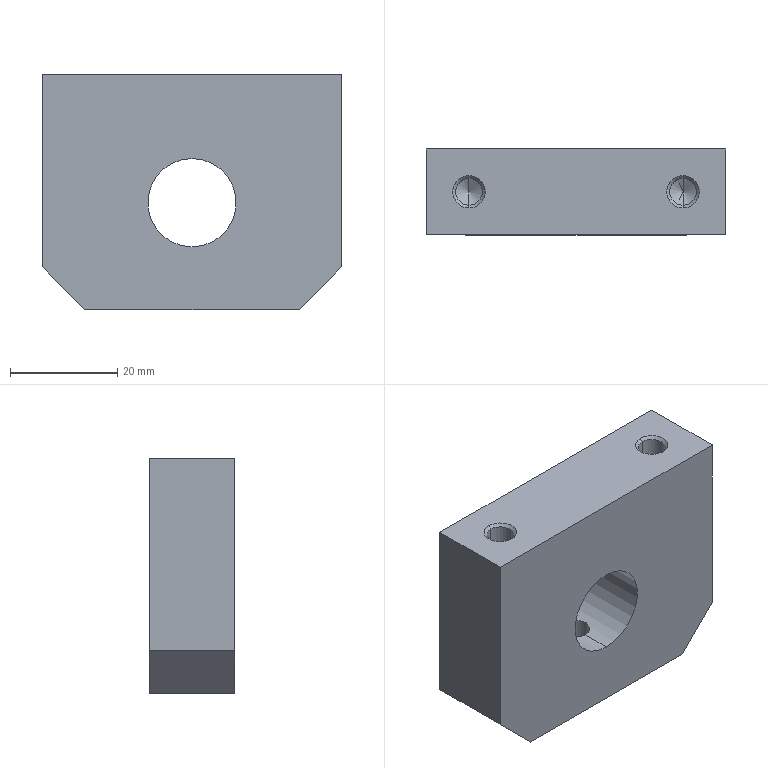Component | SolidWorks | GuideRodMount-2 | 1 solid | 26 faces | box 56 x 16 x 44 mm | volume 34052 mm3 | cone 10 | cylinder 8 | plane 8 | commonest cylinder face diameters 5 x6 16.5 x2
build123d program:
from build123d import *

# Parameters (mm, degrees)
SKETCH1_W                     = 44
SKETCH1_H                     = 56
BOSS_EXTRUDE1_DEPTH           = 16
F_16_5_16_5_DIAMETER_HOLE1_D  = 16.5
F_5_0_5_DIAMETER_HOLE1_REACH  = 54.764
F_5_0_5_DIAMETER_HOLE1_BORE_R = 2.5
F_5_0_5_DIAMETER_HOLE2_D      = 5
F_5_0_5_DIAMETER_HOLE2_DEPTH  = 17
F_5_0_5_DIAMETER_HOLE2_TIP    = 1.502
CHAMFER1_SIZE                 = 0.525
CHAMFER2_SIZE                 = 8


with BuildPart() as part:
    # Sketch1 → Boss-Extrude1 (new body)
    with BuildSketch(Plane(origin=(0, 0, -8), x_dir=(-1, 0, 0), z_dir=(0, 0, -1))):
        with Locations((-22, 0)):
            Rectangle(SKETCH1_W, SKETCH1_H)
    extrude(amount=-BOSS_EXTRUDE1_DEPTH)

    # 16.5 _16.5_ Diameter Hole1 (through all)
    with Locations(Plane.XY.offset(8)):
        with Locations((24, 0)):
            Hole(F_16_5_16_5_DIAMETER_HOLE1_D / 2)

    # 5.0 _5_ Diameter Hole1 bore → 5.0 _5_ Diameter Hole1 (cut, up to next)
    with BuildSketch(Plane(origin=(44, 0, 0), x_dir=(0, 0, -1), z_dir=(1, 0, 0)), mode=Mode.PRIVATE) as f_5_0_5_diameter_hole1_sk1:
        Circle(F_5_0_5_DIAMETER_HOLE1_BORE_R)
    f_5_0_5_diameter_hole1_tool1 = extrude(f_5_0_5_diameter_hole1_sk1.sketch, amount=-F_5_0_5_DIAMETER_HOLE1_REACH, mode=Mode.PRIVATE) & part.part
    add(f_5_0_5_diameter_hole1_tool1.solids().sort_by_distance((44, 0, 0))[0], mode=Mode.SUBTRACT)

    # 5.0 _5_ Diameter Hole2
    with Locations(Plane.ZY):
        with Locations((0, -20), (0, 20)):
            Hole(F_5_0_5_DIAMETER_HOLE2_D / 2, depth=F_5_0_5_DIAMETER_HOLE2_DEPTH)
            with Locations((0, 0, -(F_5_0_5_DIAMETER_HOLE2_DEPTH + F_5_0_5_DIAMETER_HOLE2_TIP / 2))):  # 118° drill point
                Cone(0, F_5_0_5_DIAMETER_HOLE2_D / 2, F_5_0_5_DIAMETER_HOLE2_TIP, mode=Mode.SUBTRACT)

    # Chamfer1
    chamfer1_edges = [part.edges().sort_by_distance(p)[0] for p in [
        (44, 0, 2.5),
        (0, 20, 2.5),
        (0, -20, 2.5),
    ]]
    chamfer(chamfer1_edges, length=CHAMFER1_SIZE)

    # Chamfer2
    chamfer2_edges = [part.edges().sort_by_distance(p)[0] for p in [
        (44, -28, 0),
        (44, 28, 0),
    ]]
    chamfer(chamfer2_edges, length=CHAMFER2_SIZE)


solid = part.part

# Placed as in the assembly
solid = solid.moved(Location((-36, -107, 262.5), (90, 0, -90)))
STEP:
#1=CARTESIAN_POINT('',(-0.6299,-4.114,10.314));
#2=VERTEX_POINT('',#1);
#3=CARTESIAN_POINT('',(-0.6299,-4.311,10.314));
#4=VERTEX_POINT('',#3);
#5=CARTESIAN_POINT('',(-0.6299,-4.213,10.314));
#6=DIRECTION('',(-0.,-0.,1.));
#7=DIRECTION('',(0.,-1.,0.));
#8=AXIS2_PLACEMENT_3D('',#5,#6,#7);
#9=CIRCLE('',#8,0.09843);
#10=EDGE_CURVE('',#2,#4,#9,.T.);
#11=ORIENTED_EDGE('',*,*,#10,.F.);
#12=CARTESIAN_POINT('',(-0.6299,-4.094,10.335));
#13=VERTEX_POINT('',#12);
#14=CARTESIAN_POINT('',(-0.6299,-4.114,10.314));
#15=DIRECTION('',(0.,0.7071,0.7071));
#16=VECTOR('',#15,39.37);
#17=LINE('',#14,#16);
#18=EDGE_CURVE('',#2,#13,#17,.T.);
#19=ORIENTED_EDGE('',*,*,#18,.T.);
#20=CARTESIAN_POINT('',(-0.6299,-4.332,10.335));
#21=VERTEX_POINT('',#20);
#22=CARTESIAN_POINT('',(-0.6299,-4.213,10.335));
#23=DIRECTION('',(0.,0.,-1.));
#24=DIRECTION('',(-1.,0.,0.));
#25=AXIS2_PLACEMENT_3D('',#22,#23,#24);
#26=CIRCLE('',#25,0.1191);
#27=EDGE_CURVE('',#21,#13,#26,.T.);
#28=ORIENTED_EDGE('',*,*,#27,.F.);
#29=CARTESIAN_POINT('',(-0.6299,-4.311,10.314));
#30=DIRECTION('',(0.,-0.7071,0.7071));
#31=VECTOR('',#30,39.37);
#32=LINE('',#29,#31);
#33=EDGE_CURVE('',#4,#21,#32,.T.);
#34=ORIENTED_EDGE('',*,*,#33,.F.);
#35=EDGE_LOOP('',(#11,#19,#28,#34));
#36=FACE_OUTER_BOUND('',#35,.T.);
#37=CARTESIAN_POINT('',(-0.6299,-4.213,10.314));
#38=DIRECTION('',(-0.,-0.,1.));
#39=DIRECTION('',(0.,-1.,0.));
#40=AXIS2_PLACEMENT_3D('',#37,#38,#39);
#41=CONICAL_SURFACE('',#40,0.09843,0.7854);
#42=ADVANCED_FACE('',(#36),#41,.F.);
#43=CARTESIAN_POINT('',(-2.205,-4.114,10.314));
#44=VERTEX_POINT('',#43);
#45=CARTESIAN_POINT('',(-2.205,-4.311,10.314));
#46=VERTEX_POINT('',#45);
#47=CARTESIAN_POINT('',(-2.205,-4.213,10.314));
#48=DIRECTION('',(-0.,-0.,1.));
#49=DIRECTION('',(0.,-1.,0.));
#50=AXIS2_PLACEMENT_3D('',#47,#48,#49);
#51=CIRCLE('',#50,0.09843);
#52=EDGE_CURVE('',#44,#46,#51,.T.);
#53=ORIENTED_EDGE('',*,*,#52,.F.);
#54=CARTESIAN_POINT('',(-2.205,-4.094,10.335));
#55=VERTEX_POINT('',#54);
#56=CARTESIAN_POINT('',(-2.205,-4.114,10.314));
#57=DIRECTION('',(0.,0.7071,0.7071));
#58=VECTOR('',#57,39.37);
#59=LINE('',#56,#58);
#60=EDGE_CURVE('',#44,#55,#59,.T.);
#61=ORIENTED_EDGE('',*,*,#60,.T.);
#62=CARTESIAN_POINT('',(-2.205,-4.332,10.335));
#63=VERTEX_POINT('',#62);
#64=CARTESIAN_POINT('',(-2.205,-4.213,10.335));
#65=DIRECTION('',(0.,0.,-1.));
#66=DIRECTION('',(-1.,0.,0.));
#67=AXIS2_PLACEMENT_3D('',#64,#65,#66);
#68=CIRCLE('',#67,0.1191);
#69=EDGE_CURVE('',#63,#55,#68,.T.);
#70=ORIENTED_EDGE('',*,*,#69,.F.);
#71=CARTESIAN_POINT('',(-2.205,-4.311,10.314));
#72=DIRECTION('',(0.,-0.7071,0.7071));
#73=VECTOR('',#72,39.37);
#74=LINE('',#71,#73);
#75=EDGE_CURVE('',#46,#63,#74,.T.);
#76=ORIENTED_EDGE('',*,*,#75,.F.);
#77=EDGE_LOOP('',(#53,#61,#70,#76));
#78=FACE_OUTER_BOUND('',#77,.T.);
#79=CARTESIAN_POINT('',(-2.205,-4.213,10.314));
#80=DIRECTION('',(-0.,-0.,1.));
#81=DIRECTION('',(0.,-1.,0.));
#82=AXIS2_PLACEMENT_3D('',#79,#80,#81);
#83=CONICAL_SURFACE('',#82,0.09843,0.7854);
#84=ADVANCED_FACE('',(#78),#83,.F.);
#85=CARTESIAN_POINT('',(-1.417,-4.311,8.623));
#86=VERTEX_POINT('',#85);
#87=CARTESIAN_POINT('',(-1.417,-4.114,8.623));
#88=VERTEX_POINT('',#87);
#89=CARTESIAN_POINT('',(-1.417,-4.213,8.623));
#90=DIRECTION('',(0.,0.,-1.));
#91=DIRECTION('',(0.,1.,0.));
#92=AXIS2_PLACEMENT_3D('',#89,#90,#91);
#93=CIRCLE('',#92,0.09843);
#94=EDGE_CURVE('',#86,#88,#93,.T.);
#95=ORIENTED_EDGE('',*,*,#94,.F.);
#96=CARTESIAN_POINT('',(-1.417,-4.332,8.602));
#97=VERTEX_POINT('',#96);
#98=CARTESIAN_POINT('',(-1.417,-4.311,8.623));
#99=DIRECTION('',(0.,-0.7071,-0.7071));
#100=VECTOR('',#99,39.37);
#101=LINE('',#98,#100);
#102=EDGE_CURVE('',#86,#97,#101,.T.);
#103=ORIENTED_EDGE('',*,*,#102,.T.);
#104=CARTESIAN_POINT('',(-1.417,-4.094,8.602));
#105=VERTEX_POINT('',#104);
#106=CARTESIAN_POINT('',(-1.417,-4.213,8.602));
#107=DIRECTION('',(-0.,-0.,1.));
#108=DIRECTION('',(0.,1.,0.));
#109=AXIS2_PLACEMENT_3D('',#106,#107,#108);
#110=CIRCLE('',#109,0.1191);
#111=EDGE_CURVE('',#105,#97,#110,.T.);
#112=ORIENTED_EDGE('',*,*,#111,.F.);
#113=CARTESIAN_POINT('',(-1.417,-4.114,8.623));
#114=DIRECTION('',(-0.,0.7071,-0.7071));
#115=VECTOR('',#114,39.37);
#116=LINE('',#113,#115);
#117=EDGE_CURVE('',#88,#105,#116,.T.);
#118=ORIENTED_EDGE('',*,*,#117,.F.);
#119=EDGE_LOOP('',(#95,#103,#112,#118));
#120=FACE_OUTER_BOUND('',#119,.T.);
#121=CARTESIAN_POINT('',(-1.417,-4.213,8.623));
#122=DIRECTION('',(0.,0.,-1.));
#123=DIRECTION('',(0.,1.,0.));
#124=AXIS2_PLACEMENT_3D('',#121,#122,#123);
#125=CONICAL_SURFACE('',#124,0.09843,0.7854);
#126=ADVANCED_FACE('',(#120),#125,.F.);
#127=CARTESIAN_POINT('',(-2.205,-4.114,9.665));
#128=VERTEX_POINT('',#127);
#129=CARTESIAN_POINT('',(-2.205,-4.311,9.665));
#130=VERTEX_POINT('',#129);
#131=CARTESIAN_POINT('',(-2.205,-4.213,9.665));
#132=DIRECTION('',(-0.,-0.,1.));
#133=DIRECTION('',(0.,-1.,0.));
#134=AXIS2_PLACEMENT_3D('',#131,#132,#133);
#135=CIRCLE('',#134,0.09843);
#136=EDGE_CURVE('',#128,#130,#135,.T.);
#137=ORIENTED_EDGE('',*,*,#136,.F.);
#138=CARTESIAN_POINT('',(-2.205,-4.114,10.335));
#139=DIRECTION('',(-0.,-0.,1.));
#140=VECTOR('',#139,39.37);
#141=LINE('',#138,#140);
#142=EDGE_CURVE('',#128,#44,#141,.T.);
#143=ORIENTED_EDGE('',*,*,#142,.T.);
#144=ORIENTED_EDGE('',*,*,#52,.T.);
#145=CARTESIAN_POINT('',(-2.205,-4.311,10.335));
#146=DIRECTION('',(-0.,-0.,1.));
#147=VECTOR('',#146,39.37);
#148=LINE('',#145,#147);
#149=EDGE_CURVE('',#130,#46,#148,.T.);
#150=ORIENTED_EDGE('',*,*,#149,.F.);
#151=EDGE_LOOP('',(#137,#143,#144,#150));
#152=FACE_OUTER_BOUND('',#151,.T.);
#153=CARTESIAN_POINT('',(-2.205,-4.213,10.335));
#154=DIRECTION('',(-0.,-0.,1.));
#155=DIRECTION('',(0.,-1.,0.));
#156=AXIS2_PLACEMENT_3D('',#153,#154,#155);
#157=CYLINDRICAL_SURFACE('',#156,0.09843);
#158=ADVANCED_FACE('',(#152),#157,.F.);
#159=CARTESIAN_POINT('',(-2.205,-4.213,9.606));
#160=VERTEX_POINT('',#159);
#161=CARTESIAN_POINT('',(-2.205,-4.311,9.665));
#162=DIRECTION('',(0.,-0.8572,0.515));
#163=VECTOR('',#162,39.37);
#164=LINE('',#161,#163);
#165=EDGE_CURVE('',#160,#130,#164,.T.);
#166=ORIENTED_EDGE('',*,*,#165,.F.);
#167=CARTESIAN_POINT('',(-2.205,-4.114,9.665));
#168=DIRECTION('',(0.,0.8572,0.515));
#169=VECTOR('',#168,39.37);
#170=LINE('',#167,#169);
#171=EDGE_CURVE('',#160,#128,#170,.T.);
#172=ORIENTED_EDGE('',*,*,#171,.T.);
#173=ORIENTED_EDGE('',*,*,#136,.T.);
#174=EDGE_LOOP('',(#166,#172,#173));
#175=FACE_OUTER_BOUND('',#174,.T.);
#176=CARTESIAN_POINT('',(-2.205,-4.213,9.665));
#177=DIRECTION('',(-0.,-0.,1.));
#178=DIRECTION('',(0.,-1.,0.));
#179=AXIS2_PLACEMENT_3D('',#176,#177,#178);
#180=CONICAL_SURFACE('',#179,0.09843,1.03);
#181=ADVANCED_FACE('',(#175),#180,.F.);
#182=CARTESIAN_POINT('',(-0.6299,-4.114,9.665));
#183=VERTEX_POINT('',#182);
#184=CARTESIAN_POINT('',(-0.6299,-4.311,9.665));
#185=VERTEX_POINT('',#184);
#186=CARTESIAN_POINT('',(-0.6299,-4.213,9.665));
#187=DIRECTION('',(-0.,-0.,1.));
#188=DIRECTION('',(0.,-1.,0.));
#189=AXIS2_PLACEMENT_3D('',#186,#187,#188);
#190=CIRCLE('',#189,0.09843);
#191=EDGE_CURVE('',#183,#185,#190,.T.);
#192=ORIENTED_EDGE('',*,*,#191,.F.);
#193=CARTESIAN_POINT('',(-0.6299,-4.114,10.335));
#194=DIRECTION('',(-0.,-0.,1.));
#195=VECTOR('',#194,39.37);
#196=LINE('',#193,#195);
#197=EDGE_CURVE('',#183,#2,#196,.T.);
#198=ORIENTED_EDGE('',*,*,#197,.T.);
#199=ORIENTED_EDGE('',*,*,#10,.T.);
#200=CARTESIAN_POINT('',(-0.6299,-4.311,10.335));
#201=DIRECTION('',(-0.,-0.,1.));
#202=VECTOR('',#201,39.37);
#203=LINE('',#200,#202);
#204=EDGE_CURVE('',#185,#4,#203,.T.);
#205=ORIENTED_EDGE('',*,*,#204,.F.);
#206=EDGE_LOOP('',(#192,#198,#199,#205));
#207=FACE_OUTER_BOUND('',#206,.T.);
#208=CARTESIAN_POINT('',(-0.6299,-4.213,10.335));
#209=DIRECTION('',(-0.,-0.,1.));
#210=DIRECTION('',(0.,-1.,0.));
#211=AXIS2_PLACEMENT_3D('',#208,#209,#210);
#212=CYLINDRICAL_SURFACE('',#211,0.09843);
#213=ADVANCED_FACE('',(#207),#212,.F.);
#214=CARTESIAN_POINT('',(-0.6299,-4.213,9.606));
#215=VERTEX_POINT('',#214);
#216=CARTESIAN_POINT('',(-0.6299,-4.311,9.665));
#217=DIRECTION('',(0.,-0.8572,0.515));
#218=VECTOR('',#217,39.37);
#219=LINE('',#216,#218);
#220=EDGE_CURVE('',#215,#185,#219,.T.);
#221=ORIENTED_EDGE('',*,*,#220,.F.);
#222=CARTESIAN_POINT('',(-0.6299,-4.114,9.665));
#223=DIRECTION('',(0.,0.8572,0.515));
#224=VECTOR('',#223,39.37);
#225=LINE('',#222,#224);
#226=EDGE_CURVE('',#215,#183,#225,.T.);
#227=ORIENTED_EDGE('',*,*,#226,.T.);
#228=ORIENTED_EDGE('',*,*,#191,.T.);
#229=EDGE_LOOP('',(#221,#227,#228));
#230=FACE_OUTER_BOUND('',#229,.T.);
#231=CARTESIAN_POINT('',(-0.6299,-4.213,9.665));
#232=DIRECTION('',(-0.,-0.,1.));
#233=DIRECTION('',(0.,-1.,0.));
#234=AXIS2_PLACEMENT_3D('',#231,#232,#233);
#235=CONICAL_SURFACE('',#234,0.09843,1.03);
#236=ADVANCED_FACE('',(#230),#235,.F.);
#237=CARTESIAN_POINT('',(-1.417,-4.311,9.065));
#238=VERTEX_POINT('',#237);
#239=CARTESIAN_POINT('',(-1.417,-4.114,9.065));
#240=VERTEX_POINT('',#239);
#241=CARTESIAN_POINT('',(-1.417,-4.311,9.065));
#242=CARTESIAN_POINT('',(-1.43,-4.311,9.065));
#243=CARTESIAN_POINT('',(-1.443,-4.308,9.066));
#244=CARTESIAN_POINT('',(-1.461,-4.301,9.068));
#245=CARTESIAN_POINT('',(-1.467,-4.298,9.069));
#246=CARTESIAN_POINT('',(-1.477,-4.291,9.071));
#247=CARTESIAN_POINT('',(-1.482,-4.287,9.072));
#248=CARTESIAN_POINT('',(-1.491,-4.278,9.073));
#249=CARTESIAN_POINT('',(-1.496,-4.273,9.075));
#250=CARTESIAN_POINT('',(-1.503,-4.262,9.076));
#251=CARTESIAN_POINT('',(-1.506,-4.256,9.077));
#252=CARTESIAN_POINT('',(-1.511,-4.244,9.079));
#253=CARTESIAN_POINT('',(-1.513,-4.238,9.079));
#254=CARTESIAN_POINT('',(-1.515,-4.226,9.08));
#255=CARTESIAN_POINT('',(-1.516,-4.219,9.08));
#256=CARTESIAN_POINT('',(-1.516,-4.206,9.08));
#257=CARTESIAN_POINT('',(-1.515,-4.2,9.08));
#258=CARTESIAN_POINT('',(-1.513,-4.187,9.079));
#259=CARTESIAN_POINT('',(-1.511,-4.181,9.079));
#260=CARTESIAN_POINT('',(-1.503,-4.163,9.076));
#261=CARTESIAN_POINT('',(-1.496,-4.152,9.074));
#262=CARTESIAN_POINT('',(-1.482,-4.139,9.072));
#263=CARTESIAN_POINT('',(-1.477,-4.134,9.071));
#264=CARTESIAN_POINT('',(-1.467,-4.127,9.069));
#265=CARTESIAN_POINT('',(-1.461,-4.124,9.068));
#266=CARTESIAN_POINT('',(-1.449,-4.119,9.066));
#267=CARTESIAN_POINT('',(-1.443,-4.117,9.066));
#268=CARTESIAN_POINT('',(-1.43,-4.115,9.065));
#269=CARTESIAN_POINT('',(-1.424,-4.114,9.065));
#270=CARTESIAN_POINT('',(-1.417,-4.114,9.065));
#271=B_SPLINE_CURVE_WITH_KNOTS('',3,(#241,#242,#243,#244,#245,#246,#247,#248,#249,#250,#251,#252,#253,#254,#255,#256,#257,#258,#259,#260,#261,#262,#263,#264,#265,#266,#267,#268,#269,#270),.UNSPECIFIED.,.F.,.F.,(4,2,2,2,2,2,2,2,2,2,2,2,2,2,4),(0.007863,0.008845,0.009336,0.009828,0.01032,0.01081,0.0113,0.01179,0.01228,0.01278,0.01376,0.01425,0.01474,0.01523,0.01572),.UNSPECIFIED.);
#272=EDGE_CURVE('',#238,#240,#271,.T.);
#273=ORIENTED_EDGE('',*,*,#272,.F.);
#274=CARTESIAN_POINT('',(-1.417,-4.311,8.602));
#275=DIRECTION('',(0.,0.,-1.));
#276=VECTOR('',#275,39.37);
#277=LINE('',#274,#276);
#278=EDGE_CURVE('',#238,#86,#277,.T.);
#279=ORIENTED_EDGE('',*,*,#278,.T.);
#280=ORIENTED_EDGE('',*,*,#94,.T.);
#281=CARTESIAN_POINT('',(-1.417,-4.114,8.602));
#282=DIRECTION('',(0.,0.,-1.));
#283=VECTOR('',#282,39.37);
#284=LINE('',#281,#283);
#285=EDGE_CURVE('',#240,#88,#284,.T.);
#286=ORIENTED_EDGE('',*,*,#285,.F.);
#287=EDGE_LOOP('',(#273,#279,#280,#286));
#288=FACE_OUTER_BOUND('',#287,.T.);
#289=CARTESIAN_POINT('',(-1.417,-4.213,8.602));
#290=DIRECTION('',(0.,0.,-1.));
#291=DIRECTION('',(0.,1.,0.));
#292=AXIS2_PLACEMENT_3D('',#289,#290,#291);
#293=CYLINDRICAL_SURFACE('',#292,0.09843);
#294=ADVANCED_FACE('',(#288),#293,.F.);
#295=CARTESIAN_POINT('',(-1.417,-3.898,9.715));
#296=VERTEX_POINT('',#295);
#297=CARTESIAN_POINT('',(-1.417,-3.898,9.065));
#298=VERTEX_POINT('',#297);
#299=CARTESIAN_POINT('',(-1.417,-3.898,9.39));
#300=DIRECTION('',(0.,-1.,0.));
#301=DIRECTION('',(0.,0.,-1.));
#302=AXIS2_PLACEMENT_3D('',#299,#300,#301);
#303=CIRCLE('',#302,0.3248);
#304=EDGE_CURVE('',#296,#298,#303,.T.);
#305=ORIENTED_EDGE('',*,*,#304,.F.);
#306=CARTESIAN_POINT('',(-1.417,-4.528,9.715));
#307=VERTEX_POINT('',#306);
#308=CARTESIAN_POINT('',(-1.417,-4.528,9.715));
#309=DIRECTION('',(0.,-1.,0.));
#310=VECTOR('',#309,39.37);
#311=LINE('',#308,#310);
#312=EDGE_CURVE('',#296,#307,#311,.T.);
#313=ORIENTED_EDGE('',*,*,#312,.T.);
#314=CARTESIAN_POINT('',(-1.417,-4.528,9.065));
#315=VERTEX_POINT('',#314);
#316=CARTESIAN_POINT('',(-1.417,-4.528,9.39));
#317=DIRECTION('',(0.,-1.,0.));
#318=DIRECTION('',(0.,0.,-1.));
#319=AXIS2_PLACEMENT_3D('',#316,#317,#318);
#320=CIRCLE('',#319,0.3248);
#321=EDGE_CURVE('',#307,#315,#320,.T.);
#322=ORIENTED_EDGE('',*,*,#321,.T.);
#323=CARTESIAN_POINT('',(-1.417,-4.528,9.065));
#324=DIRECTION('',(0.,-1.,0.));
#325=VECTOR('',#324,39.37);
#326=LINE('',#323,#325);
#327=EDGE_CURVE('',#238,#315,#326,.T.);
#328=ORIENTED_EDGE('',*,*,#327,.F.);
#329=ORIENTED_EDGE('',*,*,#272,.T.);
#330=CARTESIAN_POINT('',(-1.417,-4.528,9.065));
#331=DIRECTION('',(0.,-1.,0.));
#332=VECTOR('',#331,39.37);
#333=LINE('',#330,#332);
#334=EDGE_CURVE('',#298,#240,#333,.T.);
#335=ORIENTED_EDGE('',*,*,#334,.F.);
#336=EDGE_LOOP('',(#305,#313,#322,#328,#329,#335));
#337=FACE_OUTER_BOUND('',#336,.T.);
#338=CARTESIAN_POINT('',(-1.417,-4.528,9.39));
#339=DIRECTION('',(0.,-1.,0.));
#340=DIRECTION('',(0.,0.,-1.));
#341=AXIS2_PLACEMENT_3D('',#338,#339,#340);
#342=CYLINDRICAL_SURFACE('',#341,0.3248);
#343=ADVANCED_FACE('',(#337),#342,.F.);
#344=CARTESIAN_POINT('',(-0.315,-4.528,10.335));
#345=VERTEX_POINT('',#344);
#346=CARTESIAN_POINT('',(-0.315,-4.528,8.917));
#347=VERTEX_POINT('',#346);
#348=CARTESIAN_POINT('',(-0.315,-4.528,10.335));
#349=DIRECTION('',(0.,0.,-1.));
#350=VECTOR('',#349,39.37);
#351=LINE('',#348,#350);
#352=EDGE_CURVE('',#345,#347,#351,.T.);
#353=ORIENTED_EDGE('',*,*,#352,.T.);
#354=CARTESIAN_POINT('',(-0.315,-3.898,8.917));
#355=VERTEX_POINT('',#354);
#356=CARTESIAN_POINT('',(-0.315,-4.528,8.917));
#357=DIRECTION('',(-0.,1.,0.));
#358=VECTOR('',#357,39.37);
#359=LINE('',#356,#358);
#360=EDGE_CURVE('',#347,#355,#359,.T.);
#361=ORIENTED_EDGE('',*,*,#360,.T.);
#362=CARTESIAN_POINT('',(-0.315,-3.898,10.335));
#363=VERTEX_POINT('',#362);
#364=CARTESIAN_POINT('',(-0.315,-3.898,10.335));
#365=DIRECTION('',(0.,0.,-1.));
#366=VECTOR('',#365,39.37);
#367=LINE('',#364,#366);
#368=EDGE_CURVE('',#363,#355,#367,.T.);
#369=ORIENTED_EDGE('',*,*,#368,.F.);
#370=CARTESIAN_POINT('',(-0.315,-4.528,10.335));
#371=DIRECTION('',(-0.,1.,0.));
#372=VECTOR('',#371,39.37);
#373=LINE('',#370,#372);
#374=EDGE_CURVE('',#345,#363,#373,.T.);
#375=ORIENTED_EDGE('',*,*,#374,.F.);
#376=EDGE_LOOP('',(#353,#361,#369,#375));
#377=FACE_OUTER_BOUND('',#376,.T.);
#378=CARTESIAN_POINT('',(-0.315,-4.528,10.335));
#379=DIRECTION('',(1.,0.,0.));
#380=DIRECTION('',(0.,-1.,0.));
#381=AXIS2_PLACEMENT_3D('',#378,#379,#380);
#382=PLANE('',#381);
#383=ADVANCED_FACE('',(#377),#382,.T.);
#384=ORIENTED_EDGE('',*,*,#69,.T.);
#385=CARTESIAN_POINT('',(-2.205,-4.213,10.335));
#386=DIRECTION('',(0.,0.,-1.));
#387=DIRECTION('',(-1.,0.,0.));
#388=AXIS2_PLACEMENT_3D('',#385,#386,#387);
#389=CIRCLE('',#388,0.1191);
#390=EDGE_CURVE('',#55,#63,#389,.T.);
#391=ORIENTED_EDGE('',*,*,#390,.T.);
#392=EDGE_LOOP('',(#384,#391));
#393=FACE_BOUND('',#392,.T.);
#394=ORIENTED_EDGE('',*,*,#27,.T.);
#395=CARTESIAN_POINT('',(-0.6299,-4.213,10.335));
#396=DIRECTION('',(0.,0.,-1.));
#397=DIRECTION('',(-1.,0.,0.));
#398=AXIS2_PLACEMENT_3D('',#395,#396,#397);
#399=CIRCLE('',#398,0.1191);
#400=EDGE_CURVE('',#13,#21,#399,.T.);
#401=ORIENTED_EDGE('',*,*,#400,.T.);
#402=EDGE_LOOP('',(#394,#401));
#403=FACE_BOUND('',#402,.T.);
#404=CARTESIAN_POINT('',(-2.52,-3.898,10.335));
#405=VERTEX_POINT('',#404);
#406=CARTESIAN_POINT('',(-2.52,-3.898,10.335));
#407=DIRECTION('',(1.,0.,0.));
#408=VECTOR('',#407,39.37);
#409=LINE('',#406,#408);
#410=EDGE_CURVE('',#405,#363,#409,.T.);
#411=ORIENTED_EDGE('',*,*,#410,.F.);
#412=CARTESIAN_POINT('',(-2.52,-4.528,10.335));
#413=VERTEX_POINT('',#412);
#414=CARTESIAN_POINT('',(-2.52,-4.528,10.335));
#415=DIRECTION('',(-0.,1.,0.));
#416=VECTOR('',#415,39.37);
#417=LINE('',#414,#416);
#418=EDGE_CURVE('',#413,#405,#417,.T.);
#419=ORIENTED_EDGE('',*,*,#418,.F.);
#420=CARTESIAN_POINT('',(-2.52,-4.528,10.335));
#421=DIRECTION('',(1.,0.,0.));
#422=VECTOR('',#421,39.37);
#423=LINE('',#420,#422);
#424=EDGE_CURVE('',#413,#345,#423,.T.);
#425=ORIENTED_EDGE('',*,*,#424,.T.);
#426=ORIENTED_EDGE('',*,*,#374,.T.);
#427=EDGE_LOOP('',(#411,#419,#425,#426));
#428=FACE_OUTER_BOUND('',#427,.T.);
#429=CARTESIAN_POINT('',(-2.52,-4.528,10.335));
#430=DIRECTION('',(-0.,-0.,1.));
#431=DIRECTION('',(-1.,-0.,-0.));
#432=AXIS2_PLACEMENT_3D('',#429,#430,#431);
#433=PLANE('',#432);
#434=ADVANCED_FACE('',(#393,#403,#428),#433,.T.);
#435=CARTESIAN_POINT('',(-2.52,-3.898,8.917));
#436=VERTEX_POINT('',#435);
#437=CARTESIAN_POINT('',(-2.52,-3.898,8.602));
#438=DIRECTION('',(-0.,-0.,1.));
#439=VECTOR('',#438,39.37);
#440=LINE('',#437,#439);
#441=EDGE_CURVE('',#436,#405,#440,.T.);
#442=ORIENTED_EDGE('',*,*,#441,.F.);
#443=CARTESIAN_POINT('',(-2.52,-4.528,8.917));
#444=VERTEX_POINT('',#443);
#445=CARTESIAN_POINT('',(-2.52,-4.528,8.917));
#446=DIRECTION('',(0.,-1.,0.));
#447=VECTOR('',#446,39.37);
#448=LINE('',#445,#447);
#449=EDGE_CURVE('',#436,#444,#448,.T.);
#450=ORIENTED_EDGE('',*,*,#449,.T.);
#451=CARTESIAN_POINT('',(-2.52,-4.528,8.602));
#452=DIRECTION('',(-0.,-0.,1.));
#453=VECTOR('',#452,39.37);
#454=LINE('',#451,#453);
#455=EDGE_CURVE('',#444,#413,#454,.T.);
#456=ORIENTED_EDGE('',*,*,#455,.T.);
#457=ORIENTED_EDGE('',*,*,#418,.T.);
#458=EDGE_LOOP('',(#442,#450,#456,#457));
#459=FACE_OUTER_BOUND('',#458,.T.);
#460=CARTESIAN_POINT('',(-2.52,-4.528,8.602));
#461=DIRECTION('',(-1.,-0.,-0.));
#462=DIRECTION('',(-0.,1.,0.));
#463=AXIS2_PLACEMENT_3D('',#460,#461,#462);
#464=PLANE('',#463);
#465=ADVANCED_FACE('',(#459),#464,.T.);
#466=ORIENTED_EDGE('',*,*,#111,.T.);
#467=CARTESIAN_POINT('',(-1.417,-4.213,8.602));
#468=DIRECTION('',(-0.,-0.,1.));
#469=DIRECTION('',(0.,1.,0.));
#470=AXIS2_PLACEMENT_3D('',#467,#468,#469);
#471=CIRCLE('',#470,0.1191);
#472=EDGE_CURVE('',#97,#105,#471,.T.);
#473=ORIENTED_EDGE('',*,*,#472,.T.);
#474=EDGE_LOOP('',(#466,#473));
#475=FACE_BOUND('',#474,.T.);
#476=CARTESIAN_POINT('',(-0.6299,-3.898,8.602));
#477=VERTEX_POINT('',#476);
#478=CARTESIAN_POINT('',(-2.205,-3.898,8.602));
#479=VERTEX_POINT('',#478);
#480=CARTESIAN_POINT('',(-0.315,-3.898,8.602));
#481=DIRECTION('',(-1.,-0.,-0.));
#482=VECTOR('',#481,39.37);
#483=LINE('',#480,#482);
#484=EDGE_CURVE('',#477,#479,#483,.T.);
#485=ORIENTED_EDGE('',*,*,#484,.F.);
#486=CARTESIAN_POINT('',(-0.6299,-4.528,8.602));
#487=VERTEX_POINT('',#486);
#488=CARTESIAN_POINT('',(-0.6299,-4.528,8.602));
#489=DIRECTION('',(0.,-1.,0.));
#490=VECTOR('',#489,39.37);
#491=LINE('',#488,#490);
#492=EDGE_CURVE('',#477,#487,#491,.T.);
#493=ORIENTED_EDGE('',*,*,#492,.T.);
#494=CARTESIAN_POINT('',(-2.205,-4.528,8.602));
#495=VERTEX_POINT('',#494);
#496=CARTESIAN_POINT('',(-0.315,-4.528,8.602));
#497=DIRECTION('',(-1.,-0.,-0.));
#498=VECTOR('',#497,39.37);
#499=LINE('',#496,#498);
#500=EDGE_CURVE('',#487,#495,#499,.T.);
#501=ORIENTED_EDGE('',*,*,#500,.T.);
#502=CARTESIAN_POINT('',(-2.205,-4.528,8.602));
#503=DIRECTION('',(-0.,1.,0.));
#504=VECTOR('',#503,39.37);
#505=LINE('',#502,#504);
#506=EDGE_CURVE('',#495,#479,#505,.T.);
#507=ORIENTED_EDGE('',*,*,#506,.T.);
#508=EDGE_LOOP('',(#485,#493,#501,#507));
#509=FACE_OUTER_BOUND('',#508,.T.);
#510=CARTESIAN_POINT('',(-0.315,-4.528,8.602));
#511=DIRECTION('',(0.,0.,-1.));
#512=DIRECTION('',(-0.,1.,0.));
#513=AXIS2_PLACEMENT_3D('',#510,#511,#512);
#514=PLANE('',#513);
#515=ADVANCED_FACE('',(#475,#509),#514,.T.);
#516=CARTESIAN_POINT('',(-1.417,-4.528,9.39));
#517=DIRECTION('',(0.,-1.,0.));
#518=DIRECTION('',(0.,0.,-1.));
#519=AXIS2_PLACEMENT_3D('',#516,#517,#518);
#520=CIRCLE('',#519,0.3248);
#521=EDGE_CURVE('',#315,#307,#520,.T.);
#522=ORIENTED_EDGE('',*,*,#521,.F.);
#523=ORIENTED_EDGE('',*,*,#321,.F.);
#524=EDGE_LOOP('',(#522,#523));
#525=FACE_BOUND('',#524,.T.);
#526=ORIENTED_EDGE('',*,*,#500,.F.);
#527=CARTESIAN_POINT('',(-0.315,-4.528,8.917));
#528=DIRECTION('',(0.7071,0.,0.7071));
#529=VECTOR('',#528,39.37);
#530=LINE('',#527,#529);
#531=EDGE_CURVE('',#487,#347,#530,.T.);
#532=ORIENTED_EDGE('',*,*,#531,.T.);
#533=ORIENTED_EDGE('',*,*,#352,.F.);
#534=ORIENTED_EDGE('',*,*,#424,.F.);
#535=ORIENTED_EDGE('',*,*,#455,.F.);
#536=CARTESIAN_POINT('',(-2.205,-4.528,8.602));
#537=DIRECTION('',(0.7071,0.,-0.7071));
#538=VECTOR('',#537,39.37);
#539=LINE('',#536,#538);
#540=EDGE_CURVE('',#444,#495,#539,.T.);
#541=ORIENTED_EDGE('',*,*,#540,.T.);
#542=EDGE_LOOP('',(#526,#532,#533,#534,#535,#541));
#543=FACE_OUTER_BOUND('',#542,.T.);
#544=CARTESIAN_POINT('',(-1.417,-4.528,10.335));
#545=DIRECTION('',(-0.,1.,0.));
#546=DIRECTION('',(-0.,-0.,1.));
#547=AXIS2_PLACEMENT_3D('',#544,#545,#546);
#548=PLANE('',#547);
#549=ADVANCED_FACE('',(#525,#543),#548,.F.);
#550=CARTESIAN_POINT('',(-1.417,-3.898,9.39));
#551=DIRECTION('',(0.,-1.,0.));
#552=DIRECTION('',(0.,0.,-1.));
#553=AXIS2_PLACEMENT_3D('',#550,#551,#552);
#554=CIRCLE('',#553,0.3248);
#555=EDGE_CURVE('',#298,#296,#554,.T.);
#556=ORIENTED_EDGE('',*,*,#555,.T.);
#557=ORIENTED_EDGE('',*,*,#304,.T.);
#558=EDGE_LOOP('',(#556,#557));
#559=FACE_BOUND('',#558,.T.);
#560=ORIENTED_EDGE('',*,*,#368,.T.);
#561=CARTESIAN_POINT('',(-0.1575,-3.898,9.075));
#562=DIRECTION('',(-0.7071,-0.,-0.7071));
#563=VECTOR('',#562,39.37);
#564=LINE('',#561,#563);
#565=EDGE_CURVE('',#355,#477,#564,.T.);
#566=ORIENTED_EDGE('',*,*,#565,.T.);
#567=ORIENTED_EDGE('',*,*,#484,.T.);
#568=CARTESIAN_POINT('',(-2.677,-3.898,9.075));
#569=DIRECTION('',(-0.7071,-0.,0.7071));
#570=VECTOR('',#569,39.37);
#571=LINE('',#568,#570);
#572=EDGE_CURVE('',#479,#436,#571,.T.);
#573=ORIENTED_EDGE('',*,*,#572,.T.);
#574=ORIENTED_EDGE('',*,*,#441,.T.);
#575=ORIENTED_EDGE('',*,*,#410,.T.);
#576=EDGE_LOOP('',(#560,#566,#567,#573,#574,#575));
#577=FACE_OUTER_BOUND('',#576,.T.);
#578=CARTESIAN_POINT('',(-1.417,-3.898,10.335));
#579=DIRECTION('',(-0.,1.,0.));
#580=DIRECTION('',(-0.,-0.,1.));
#581=AXIS2_PLACEMENT_3D('',#578,#579,#580);
#582=PLANE('',#581);
#583=ADVANCED_FACE('',(#559,#577),#582,.T.);
#584=ORIENTED_EDGE('',*,*,#312,.F.);
#585=ORIENTED_EDGE('',*,*,#555,.F.);
#586=ORIENTED_EDGE('',*,*,#334,.T.);
#587=CARTESIAN_POINT('',(-1.417,-4.114,9.065));
#588=CARTESIAN_POINT('',(-1.411,-4.114,9.065));
#589=CARTESIAN_POINT('',(-1.404,-4.115,9.065));
#590=CARTESIAN_POINT('',(-1.392,-4.117,9.066));
#591=CARTESIAN_POINT('',(-1.385,-4.119,9.066));
#592=CARTESIAN_POINT('',(-1.374,-4.124,9.068));
#593=CARTESIAN_POINT('',(-1.368,-4.127,9.069));
#594=CARTESIAN_POINT('',(-1.357,-4.134,9.071));
#595=CARTESIAN_POINT('',(-1.352,-4.139,9.072));
#596=CARTESIAN_POINT('',(-1.339,-4.152,9.074));
#597=CARTESIAN_POINT('',(-1.331,-4.163,9.076));
#598=CARTESIAN_POINT('',(-1.324,-4.181,9.079));
#599=CARTESIAN_POINT('',(-1.322,-4.187,9.079));
#600=CARTESIAN_POINT('',(-1.32,-4.2,9.08));
#601=CARTESIAN_POINT('',(-1.319,-4.206,9.08));
#602=CARTESIAN_POINT('',(-1.319,-4.219,9.08));
#603=CARTESIAN_POINT('',(-1.32,-4.226,9.08));
#604=CARTESIAN_POINT('',(-1.322,-4.238,9.079));
#605=CARTESIAN_POINT('',(-1.324,-4.244,9.079));
#606=CARTESIAN_POINT('',(-1.329,-4.256,9.077));
#607=CARTESIAN_POINT('',(-1.332,-4.262,9.076));
#608=CARTESIAN_POINT('',(-1.339,-4.273,9.075));
#609=CARTESIAN_POINT('',(-1.343,-4.278,9.073));
#610=CARTESIAN_POINT('',(-1.352,-4.287,9.072));
#611=CARTESIAN_POINT('',(-1.357,-4.291,9.071));
#612=CARTESIAN_POINT('',(-1.368,-4.298,9.069));
#613=CARTESIAN_POINT('',(-1.374,-4.301,9.068));
#614=CARTESIAN_POINT('',(-1.385,-4.306,9.066));
#615=CARTESIAN_POINT('',(-1.392,-4.308,9.066));
#616=CARTESIAN_POINT('',(-1.404,-4.31,9.065));
#617=CARTESIAN_POINT('',(-1.411,-4.311,9.065));
#618=CARTESIAN_POINT('',(-1.417,-4.311,9.065));
#619=B_SPLINE_CURVE_WITH_KNOTS('',3,(#587,#588,#589,#590,#591,#592,#593,#594,#595,#596,#597,#598,#599,#600,#601,#602,#603,#604,#605,#606,#607,#608,#609,#610,#611,#612,#613,#614,#615,#616,#617,#618),.UNSPECIFIED.,.F.,.F.,(4,2,2,2,2,2,2,2,2,2,2,2,2,2,2,4),(0.,0.0004914,0.0009828,0.001474,0.001966,0.002948,0.00344,0.003931,0.004423,0.004914,0.005406,0.005897,0.006388,0.00688,0.007371,0.007863),.UNSPECIFIED.);
#620=EDGE_CURVE('',#240,#238,#619,.T.);
#621=ORIENTED_EDGE('',*,*,#620,.T.);
#622=ORIENTED_EDGE('',*,*,#327,.T.);
#623=ORIENTED_EDGE('',*,*,#521,.T.);
#624=EDGE_LOOP('',(#584,#585,#586,#621,#622,#623));
#625=FACE_OUTER_BOUND('',#624,.T.);
#626=CARTESIAN_POINT('',(-1.417,-4.528,9.39));
#627=DIRECTION('',(0.,-1.,0.));
#628=DIRECTION('',(0.,0.,-1.));
#629=AXIS2_PLACEMENT_3D('',#626,#627,#628);
#630=CYLINDRICAL_SURFACE('',#629,0.3248);
#631=ADVANCED_FACE('',(#625),#630,.F.);
#632=ORIENTED_EDGE('',*,*,#278,.F.);
#633=ORIENTED_EDGE('',*,*,#620,.F.);
#634=ORIENTED_EDGE('',*,*,#285,.T.);
#635=CARTESIAN_POINT('',(-1.417,-4.213,8.623));
#636=DIRECTION('',(0.,0.,-1.));
#637=DIRECTION('',(0.,1.,0.));
#638=AXIS2_PLACEMENT_3D('',#635,#636,#637);
#639=CIRCLE('',#638,0.09843);
#640=EDGE_CURVE('',#88,#86,#639,.T.);
#641=ORIENTED_EDGE('',*,*,#640,.T.);
#642=EDGE_LOOP('',(#632,#633,#634,#641));
#643=FACE_OUTER_BOUND('',#642,.T.);
#644=CARTESIAN_POINT('',(-1.417,-4.213,8.602));
#645=DIRECTION('',(0.,0.,-1.));
#646=DIRECTION('',(0.,1.,0.));
#647=AXIS2_PLACEMENT_3D('',#644,#645,#646);
#648=CYLINDRICAL_SURFACE('',#647,0.09843);
#649=ADVANCED_FACE('',(#643),#648,.F.);
#650=ORIENTED_EDGE('',*,*,#226,.F.);
#651=ORIENTED_EDGE('',*,*,#220,.T.);
#652=CARTESIAN_POINT('',(-0.6299,-4.213,9.665));
#653=DIRECTION('',(-0.,-0.,1.));
#654=DIRECTION('',(0.,-1.,0.));
#655=AXIS2_PLACEMENT_3D('',#652,#653,#654);
#656=CIRCLE('',#655,0.09843);
#657=EDGE_CURVE('',#185,#183,#656,.T.);
#658=ORIENTED_EDGE('',*,*,#657,.T.);
#659=EDGE_LOOP('',(#650,#651,#658));
#660=FACE_OUTER_BOUND('',#659,.T.);
#661=CARTESIAN_POINT('',(-0.6299,-4.213,9.665));
#662=DIRECTION('',(-0.,-0.,1.));
#663=DIRECTION('',(0.,-1.,0.));
#664=AXIS2_PLACEMENT_3D('',#661,#662,#663);
#665=CONICAL_SURFACE('',#664,0.09843,1.03);
#666=ADVANCED_FACE('',(#660),#665,.F.);
#667=ORIENTED_EDGE('',*,*,#197,.F.);
#668=ORIENTED_EDGE('',*,*,#657,.F.);
#669=ORIENTED_EDGE('',*,*,#204,.T.);
#670=CARTESIAN_POINT('',(-0.6299,-4.213,10.314));
#671=DIRECTION('',(-0.,-0.,1.));
#672=DIRECTION('',(0.,-1.,0.));
#673=AXIS2_PLACEMENT_3D('',#670,#671,#672);
#674=CIRCLE('',#673,0.09843);
#675=EDGE_CURVE('',#4,#2,#674,.T.);
#676=ORIENTED_EDGE('',*,*,#675,.T.);
#677=EDGE_LOOP('',(#667,#668,#669,#676));
#678=FACE_OUTER_BOUND('',#677,.T.);
#679=CARTESIAN_POINT('',(-0.6299,-4.213,10.335));
#680=DIRECTION('',(-0.,-0.,1.));
#681=DIRECTION('',(0.,-1.,0.));
#682=AXIS2_PLACEMENT_3D('',#679,#680,#681);
#683=CYLINDRICAL_SURFACE('',#682,0.09843);
#684=ADVANCED_FACE('',(#678),#683,.F.);
#685=ORIENTED_EDGE('',*,*,#171,.F.);
#686=ORIENTED_EDGE('',*,*,#165,.T.);
#687=CARTESIAN_POINT('',(-2.205,-4.213,9.665));
#688=DIRECTION('',(-0.,-0.,1.));
#689=DIRECTION('',(0.,-1.,0.));
#690=AXIS2_PLACEMENT_3D('',#687,#688,#689);
#691=CIRCLE('',#690,0.09843);
#692=EDGE_CURVE('',#130,#128,#691,.T.);
#693=ORIENTED_EDGE('',*,*,#692,.T.);
#694=EDGE_LOOP('',(#685,#686,#693));
#695=FACE_OUTER_BOUND('',#694,.T.);
#696=CARTESIAN_POINT('',(-2.205,-4.213,9.665));
#697=DIRECTION('',(-0.,-0.,1.));
#698=DIRECTION('',(0.,-1.,0.));
#699=AXIS2_PLACEMENT_3D('',#696,#697,#698);
#700=CONICAL_SURFACE('',#699,0.09843,1.03);
#701=ADVANCED_FACE('',(#695),#700,.F.);
#702=ORIENTED_EDGE('',*,*,#142,.F.);
#703=ORIENTED_EDGE('',*,*,#692,.F.);
#704=ORIENTED_EDGE('',*,*,#149,.T.);
#705=CARTESIAN_POINT('',(-2.205,-4.213,10.314));
#706=DIRECTION('',(-0.,-0.,1.));
#707=DIRECTION('',(0.,-1.,0.));
#708=AXIS2_PLACEMENT_3D('',#705,#706,#707);
#709=CIRCLE('',#708,0.09843);
#710=EDGE_CURVE('',#46,#44,#709,.T.);
#711=ORIENTED_EDGE('',*,*,#710,.T.);
#712=EDGE_LOOP('',(#702,#703,#704,#711));
#713=FACE_OUTER_BOUND('',#712,.T.);
#714=CARTESIAN_POINT('',(-2.205,-4.213,10.335));
#715=DIRECTION('',(-0.,-0.,1.));
#716=DIRECTION('',(0.,-1.,0.));
#717=AXIS2_PLACEMENT_3D('',#714,#715,#716);
#718=CYLINDRICAL_SURFACE('',#717,0.09843);
#719=ADVANCED_FACE('',(#713),#718,.F.);
#720=ORIENTED_EDGE('',*,*,#102,.F.);
#721=ORIENTED_EDGE('',*,*,#640,.F.);
#722=ORIENTED_EDGE('',*,*,#117,.T.);
#723=ORIENTED_EDGE('',*,*,#472,.F.);
#724=EDGE_LOOP('',(#720,#721,#722,#723));
#725=FACE_OUTER_BOUND('',#724,.T.);
#726=CARTESIAN_POINT('',(-1.417,-4.213,8.623));
#727=DIRECTION('',(0.,0.,-1.));
#728=DIRECTION('',(0.,1.,0.));
#729=AXIS2_PLACEMENT_3D('',#726,#727,#728);
#730=CONICAL_SURFACE('',#729,0.09843,0.7854);
#731=ADVANCED_FACE('',(#725),#730,.F.);
#732=ORIENTED_EDGE('',*,*,#60,.F.);
#733=ORIENTED_EDGE('',*,*,#710,.F.);
#734=ORIENTED_EDGE('',*,*,#75,.T.);
#735=ORIENTED_EDGE('',*,*,#390,.F.);
#736=EDGE_LOOP('',(#732,#733,#734,#735));
#737=FACE_OUTER_BOUND('',#736,.T.);
#738=CARTESIAN_POINT('',(-2.205,-4.213,10.314));
#739=DIRECTION('',(-0.,-0.,1.));
#740=DIRECTION('',(0.,-1.,0.));
#741=AXIS2_PLACEMENT_3D('',#738,#739,#740);
#742=CONICAL_SURFACE('',#741,0.09843,0.7854);
#743=ADVANCED_FACE('',(#737),#742,.F.);
#744=ORIENTED_EDGE('',*,*,#18,.F.);
#745=ORIENTED_EDGE('',*,*,#675,.F.);
#746=ORIENTED_EDGE('',*,*,#33,.T.);
#747=ORIENTED_EDGE('',*,*,#400,.F.);
#748=EDGE_LOOP('',(#744,#745,#746,#747));
#749=FACE_OUTER_BOUND('',#748,.T.);
#750=CARTESIAN_POINT('',(-0.6299,-4.213,10.314));
#751=DIRECTION('',(-0.,-0.,1.));
#752=DIRECTION('',(0.,-1.,0.));
#753=AXIS2_PLACEMENT_3D('',#750,#751,#752);
#754=CONICAL_SURFACE('',#753,0.09843,0.7854);
#755=ADVANCED_FACE('',(#749),#754,.F.);
#756=ORIENTED_EDGE('',*,*,#531,.F.);
#757=ORIENTED_EDGE('',*,*,#492,.F.);
#758=ORIENTED_EDGE('',*,*,#565,.F.);
#759=ORIENTED_EDGE('',*,*,#360,.F.);
#760=EDGE_LOOP('',(#756,#757,#758,#759));
#761=FACE_OUTER_BOUND('',#760,.T.);
#762=CARTESIAN_POINT('',(-0.315,-4.528,8.917));
#763=DIRECTION('',(-0.7071,-0.,0.7071));
#764=DIRECTION('',(-0.,1.,0.));
#765=AXIS2_PLACEMENT_3D('',#762,#763,#764);
#766=PLANE('',#765);
#767=ADVANCED_FACE('',(#761),#766,.F.);
#768=ORIENTED_EDGE('',*,*,#540,.F.);
#769=ORIENTED_EDGE('',*,*,#449,.F.);
#770=ORIENTED_EDGE('',*,*,#572,.F.);
#771=ORIENTED_EDGE('',*,*,#506,.F.);
#772=EDGE_LOOP('',(#768,#769,#770,#771));
#773=FACE_OUTER_BOUND('',#772,.T.);
#774=CARTESIAN_POINT('',(-2.205,-4.528,8.602));
#775=DIRECTION('',(0.7071,0.,0.7071));
#776=DIRECTION('',(-0.,1.,0.));
#777=AXIS2_PLACEMENT_3D('',#774,#775,#776);
#778=PLANE('',#777);
#779=ADVANCED_FACE('',(#773),#778,.F.);
#780=CLOSED_SHELL('',(#42,#84,#126,#158,#181,#213,#236,#294,#343,#383,#434,#465,#515,#549,#583,#631,#649,#666,#684,#701,#719,#731,#743,#755,#767,#779));
#781=MANIFOLD_SOLID_BREP('',#780);
#782=CARTESIAN_POINT('',(0.,0.,0.));
#783=DIRECTION('',(0.,0.,1.));
#784=DIRECTION('',(1.,0.,0.));
#785=AXIS2_PLACEMENT_3D('',#782,#783,#784);
#786=(LENGTH_UNIT()NAMED_UNIT(*)SI_UNIT($,.METRE.));
#787=LENGTH_MEASURE_WITH_UNIT(LENGTH_MEASURE(0.0254),#786);
#788=DIMENSIONAL_EXPONENTS(1.,0.,0.,0.,0.,0.,0.);
#789=(CONVERSION_BASED_UNIT('',#787)LENGTH_UNIT()NAMED_UNIT(#788));
#790=UNCERTAINTY_MEASURE_WITH_UNIT(LENGTH_MEASURE(0.00001),#789,'','');
#791=(NAMED_UNIT(*)PLANE_ANGLE_UNIT()SI_UNIT($,.RADIAN.));
#792=(NAMED_UNIT(*)SI_UNIT($,.STERADIAN.)SOLID_ANGLE_UNIT());
#793=(GEOMETRIC_REPRESENTATION_CONTEXT(3)GLOBAL_UNCERTAINTY_ASSIGNED_CONTEXT((#790))GLOBAL_UNIT_ASSIGNED_CONTEXT((#789,#791,#792))REPRESENTATION_CONTEXT('',''));
#794=ADVANCED_BREP_SHAPE_REPRESENTATION('',(#781,#785),#793);
#795=COLOUR_RGB('',0.7922,0.8196,0.9333);
#796=FILL_AREA_STYLE_COLOUR('',#795);
#797=FILL_AREA_STYLE('',(#796));
#798=SURFACE_STYLE_FILL_AREA(#797);
#799=SURFACE_SIDE_STYLE('',(#798));
#800=SURFACE_STYLE_USAGE(.BOTH.,#799);
#801=PRESENTATION_STYLE_ASSIGNMENT((#800));
#802=STYLED_ITEM('',(#801),#781);
#803=PRESENTATION_LAYER_ASSIGNMENT('','',(#802));
#804=(LENGTH_UNIT()NAMED_UNIT(*)SI_UNIT($,.METRE.));
#805=LENGTH_MEASURE_WITH_UNIT(LENGTH_MEASURE(0.0254),#804);
#806=DIMENSIONAL_EXPONENTS(1.,0.,0.,0.,0.,0.,0.);
#807=(CONVERSION_BASED_UNIT('',#805)LENGTH_UNIT()NAMED_UNIT(#806));
#808=UNCERTAINTY_MEASURE_WITH_UNIT(LENGTH_MEASURE(0.00001),#807,'','');
#809=(NAMED_UNIT(*)PLANE_ANGLE_UNIT()SI_UNIT($,.RADIAN.));
#810=(NAMED_UNIT(*)SI_UNIT($,.STERADIAN.)SOLID_ANGLE_UNIT());
#811=(GEOMETRIC_REPRESENTATION_CONTEXT(3)GLOBAL_UNCERTAINTY_ASSIGNED_CONTEXT((#808))GLOBAL_UNIT_ASSIGNED_CONTEXT((#807,#809,#810))REPRESENTATION_CONTEXT('',''));
#812=MECHANICAL_DESIGN_GEOMETRIC_PRESENTATION_REPRESENTATION('',(#802),#811);